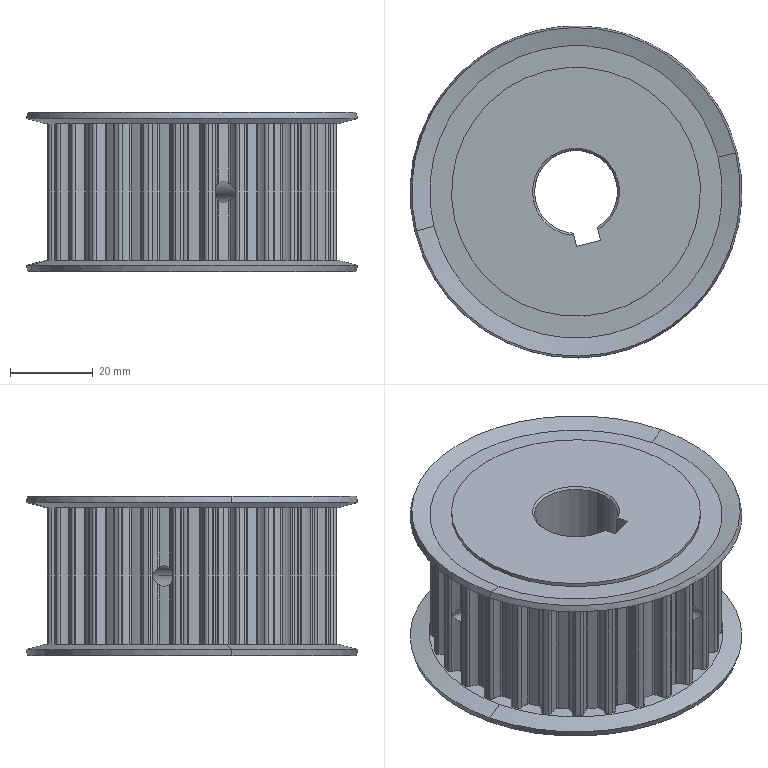Component | SolidWorks | ZDG0406-A03-B03-X1-1 | 1 solid | 295 faces | volume 122800 mm3 | cylinder 268 | cone 18 | plane 9 | commonest cylinder face diameters 0.8 x70 1.5 x68 10.6 x58 64.27 x31 69.93 x28 60 x4 4.917 x4 20 x3 | material 45#